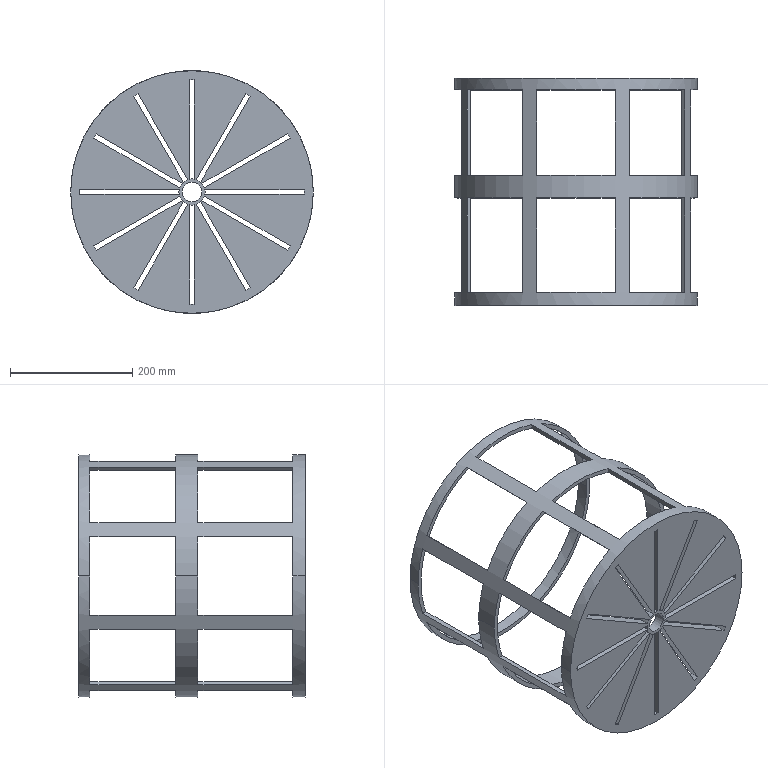Component | SolidWorks | Tray-1 | 1 solid | 123 faces | box 396.06 x 370.66 x 396.06 mm | volume 2665635 mm3 | plane 91 | cylinder 32 | commonest cylinder face diameters 42.675 x13 366.053 x13 32.237 x2 382.228 x2 396.057 x2
build123d program:
from build123d import *

# Parameters (mm, degrees)
SKETCH1_2_R                 = 198.028
SKETCH1_2_R_2               = 191.114
BOSS_EXTRUDE1_DEPTH         = 570
SKETCH2_W                   = 128.801
SKETCH2_H                   = 154.689
SKETCH2_H_2                 = 140.056
SKETCH2_H_3                 = 152.675
CUT_EXTRUDE1_DEPTH          = 172
CIRPATTERN1_COUNT           = 8
CUT_EXTRUDE2_START          = -196.337
SKETCH3_R                   = 198.028
CUT_EXTRUDE2_DEPTH          = 196.337
SKETCH4_R                   = 191.114
BOSS_EXTRUDE2_DEPTH         = 20
SKETCH5_R                   = 16.119
CUT_EXTRUDE3_DEPTH          = 152
CUT_EXTRUDE4_DEPTH          = 152
CIRPATTERN2_COUNT           = 12
SEATONSHELLFLOOR_DEPTH      = 3
SEATONSHELLFLOOR_DEPTH_BACK = 3
SKETCH1_R                   = 205


with BuildPart() as part:
    # Sketch1_2 → Boss-Extrude1 (new body)
    with BuildSketch(Plane.XY):
        with Locations(Location((-270, -250, 0), (0, 0, 270))):
            Circle(SKETCH1_2_R)
        with Locations(Location((-270, -250, 0), (0, 0, 270))):
            Circle(SKETCH1_2_R_2, mode=Mode.SUBTRACT)
    extrude(amount=BOSS_EXTRUDE1_DEPTH)

    # Sketch2 → Cut-Extrude1 (cut)
    with BuildSketch(Plane(origin=(0, 0, 0), x_dir=(1, 0, 0), z_dir=(0, 1, 0))):
        with Locations((-270, -101.253)):
            Rectangle(SKETCH2_W, SKETCH2_H)
        with Locations((-270, -285)):
            Rectangle(SKETCH2_W, SKETCH2_H_2)
        with Locations((-270, -450)):
            Rectangle(SKETCH2_W, SKETCH2_H_3)
    cut_extrude1 = extrude(amount=-CUT_EXTRUDE1_DEPTH, mode=Mode.SUBTRACT)

    # CirPattern1: Cut-Extrude1 ×8 about axis
    cirpattern1_axis = Axis((-270, -250, 0), (0, 0, 1))
    for i in range(1, CIRPATTERN1_COUNT):
        add(cut_extrude1.rotate(cirpattern1_axis, i * 360 / CIRPATTERN1_COUNT), mode=Mode.SUBTRACT)

    # Sketch3 → Cut-Extrude2 (cut)
    with BuildSketch(Plane.XY.offset(570).offset(CUT_EXTRUDE2_START)):
        with Locations(Location((-270, -250, 0), (0, 0, 180))):
            Circle(SKETCH3_R)
    extrude(amount=CUT_EXTRUDE2_DEPTH, mode=Mode.SUBTRACT)

    # Sketch4 → Boss-Extrude2 (add)
    with BuildSketch(Plane.XY):
        with Locations(Location((-270, -250, 0), (0, 0, 180))):
            Circle(SKETCH4_R)
    extrude(amount=BOSS_EXTRUDE2_DEPTH)

    # Sketch5 → Cut-Extrude3 (cut)
    with BuildSketch(Plane.XY.offset(20)):
        with Locations((-270, -250)):
            Circle(SKETCH5_R)
    extrude(amount=-CUT_EXTRUDE3_DEPTH, mode=Mode.SUBTRACT)

    # Sketch6 → Cut-Extrude4 (cut)
    with BuildSketch(Plane.XY.offset(20)):
        with BuildLine():
            Line((-452.983, -253.931), (-290.959, -253.931))
            ThreePointArc((-290.959, -253.931), (-291.338, -249.931), (-290.959, -245.931))
            Line((-290.959, -245.931), (-452.983, -245.931))
            ThreePointArc((-452.983, -245.931), (-453.026, -249.931), (-452.983, -253.931))
        make_face()
    cut_extrude4 = extrude(amount=-CUT_EXTRUDE4_DEPTH, mode=Mode.SUBTRACT)

    # CirPattern2: Cut-Extrude4 ×12 about axis
    cirpattern2_axis = Axis((-270, -250, 0), (0, 0, 1))
    for i in range(1, CIRPATTERN2_COUNT):
        add(cut_extrude4.rotate(cirpattern2_axis, i * 360 / CIRPATTERN2_COUNT), mode=Mode.SUBTRACT)

    # Sketch1 → SeatOnShellFloor (cut, two sides: drawn at the far end of the back side and taken through both)
    with BuildSketch(Plane.XY.offset(-SEATONSHELLFLOOR_DEPTH_BACK)):
        with Locations((-270, -250)):
            Circle(SKETCH1_R)
    extrude(amount=SEATONSHELLFLOOR_DEPTH + SEATONSHELLFLOOR_DEPTH_BACK, mode=Mode.SUBTRACT)


solid = part.part

# Placed as in the assembly
solid = solid.moved(Location((146.978, -378.978, -664.298), (-90, 0, 0)))